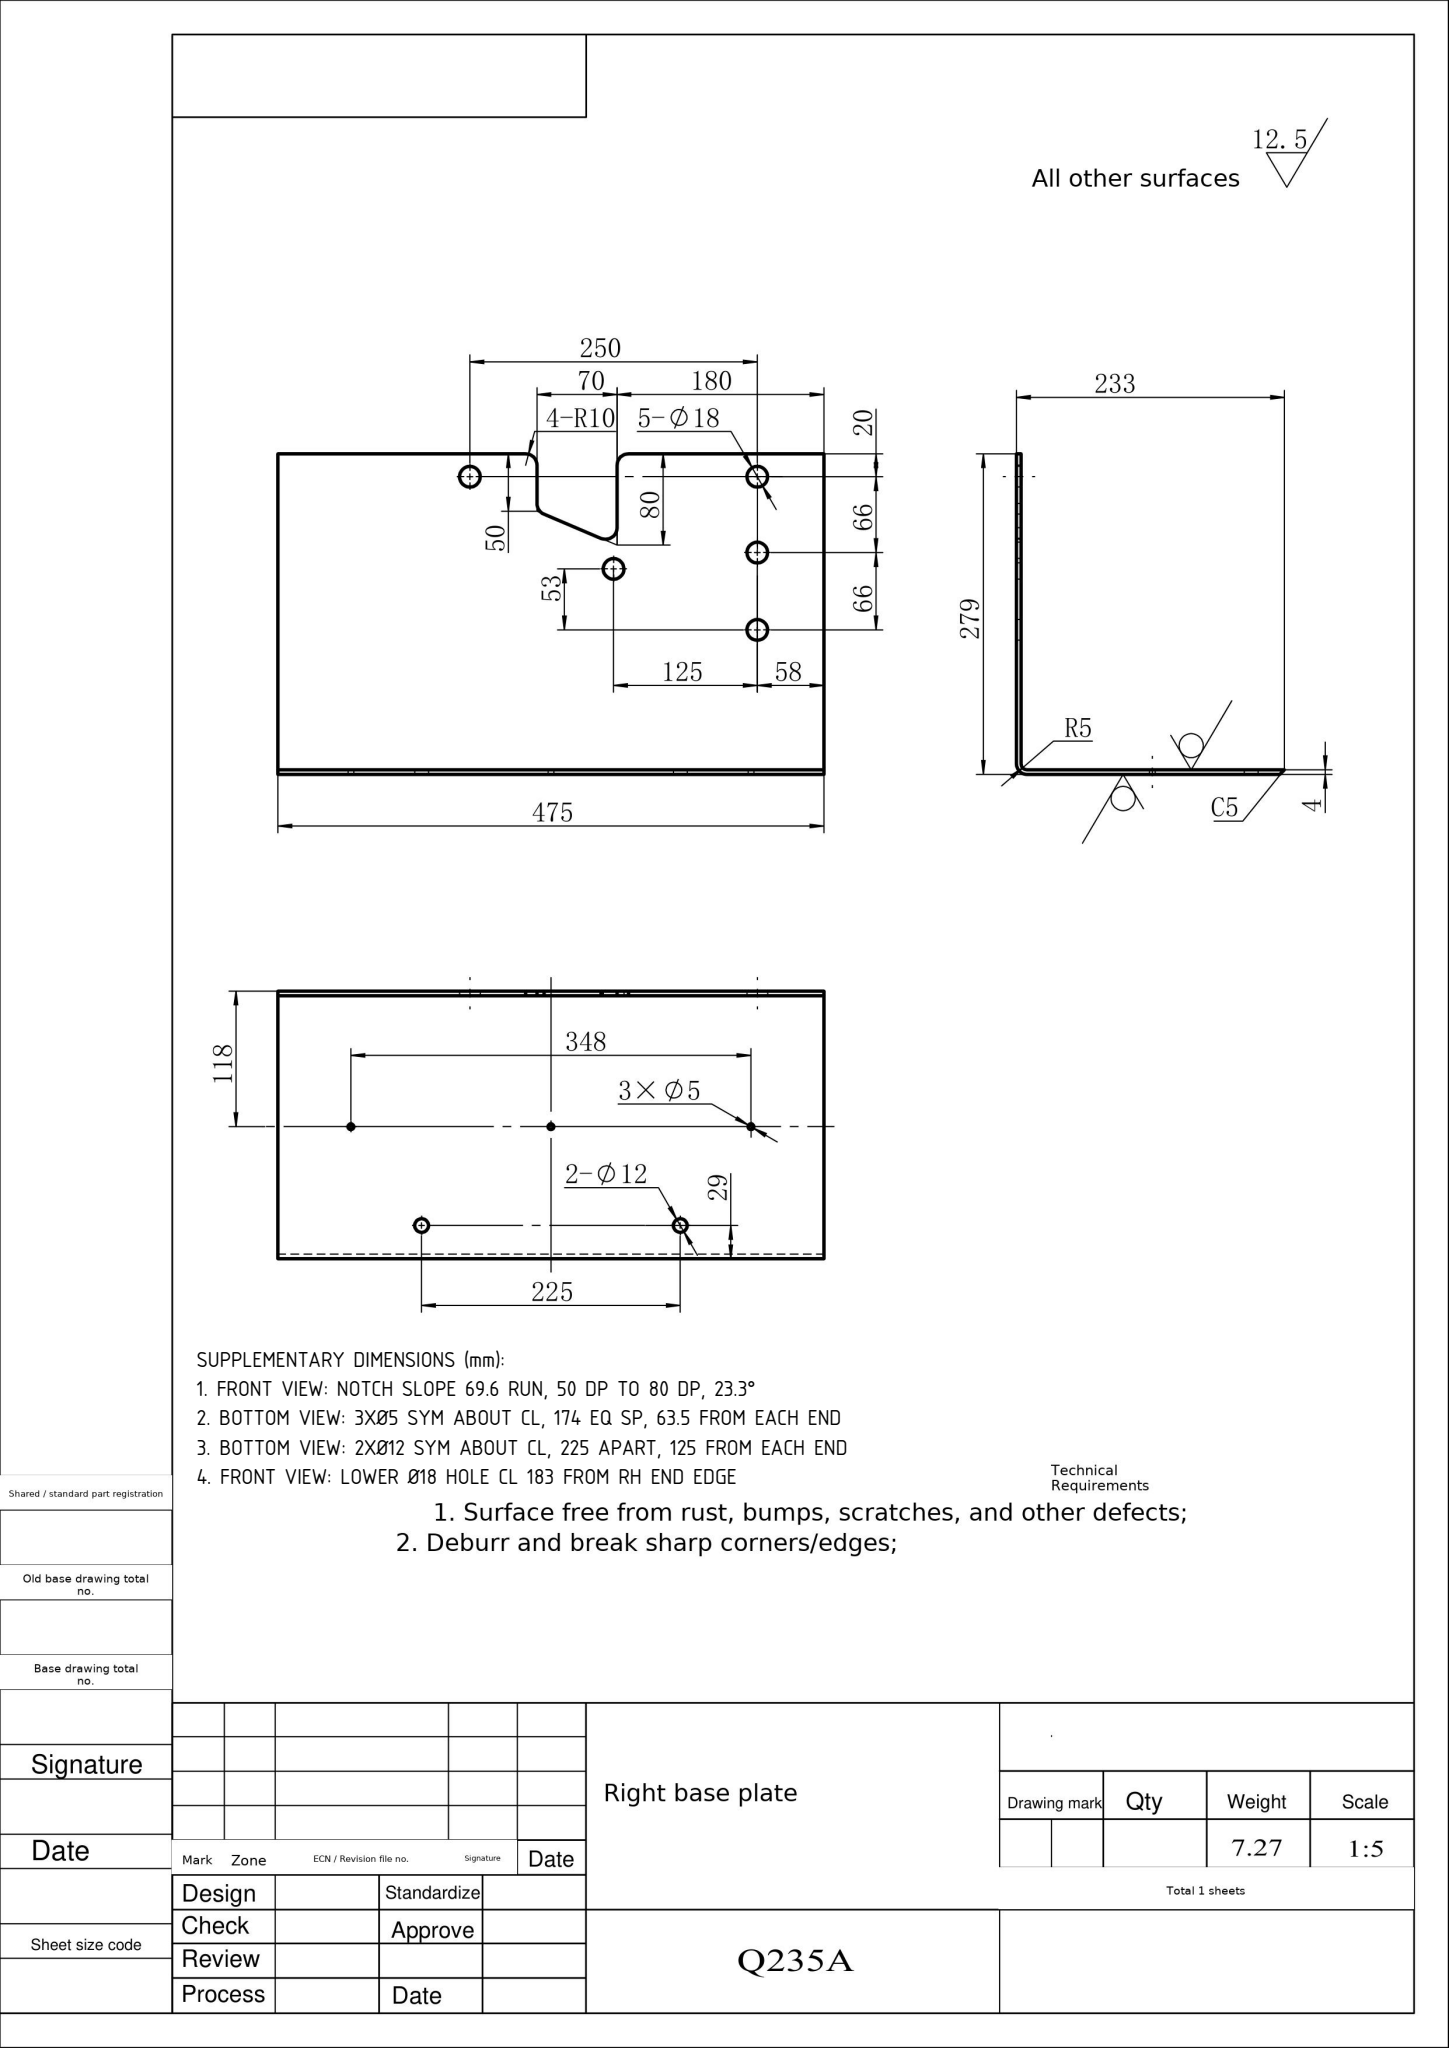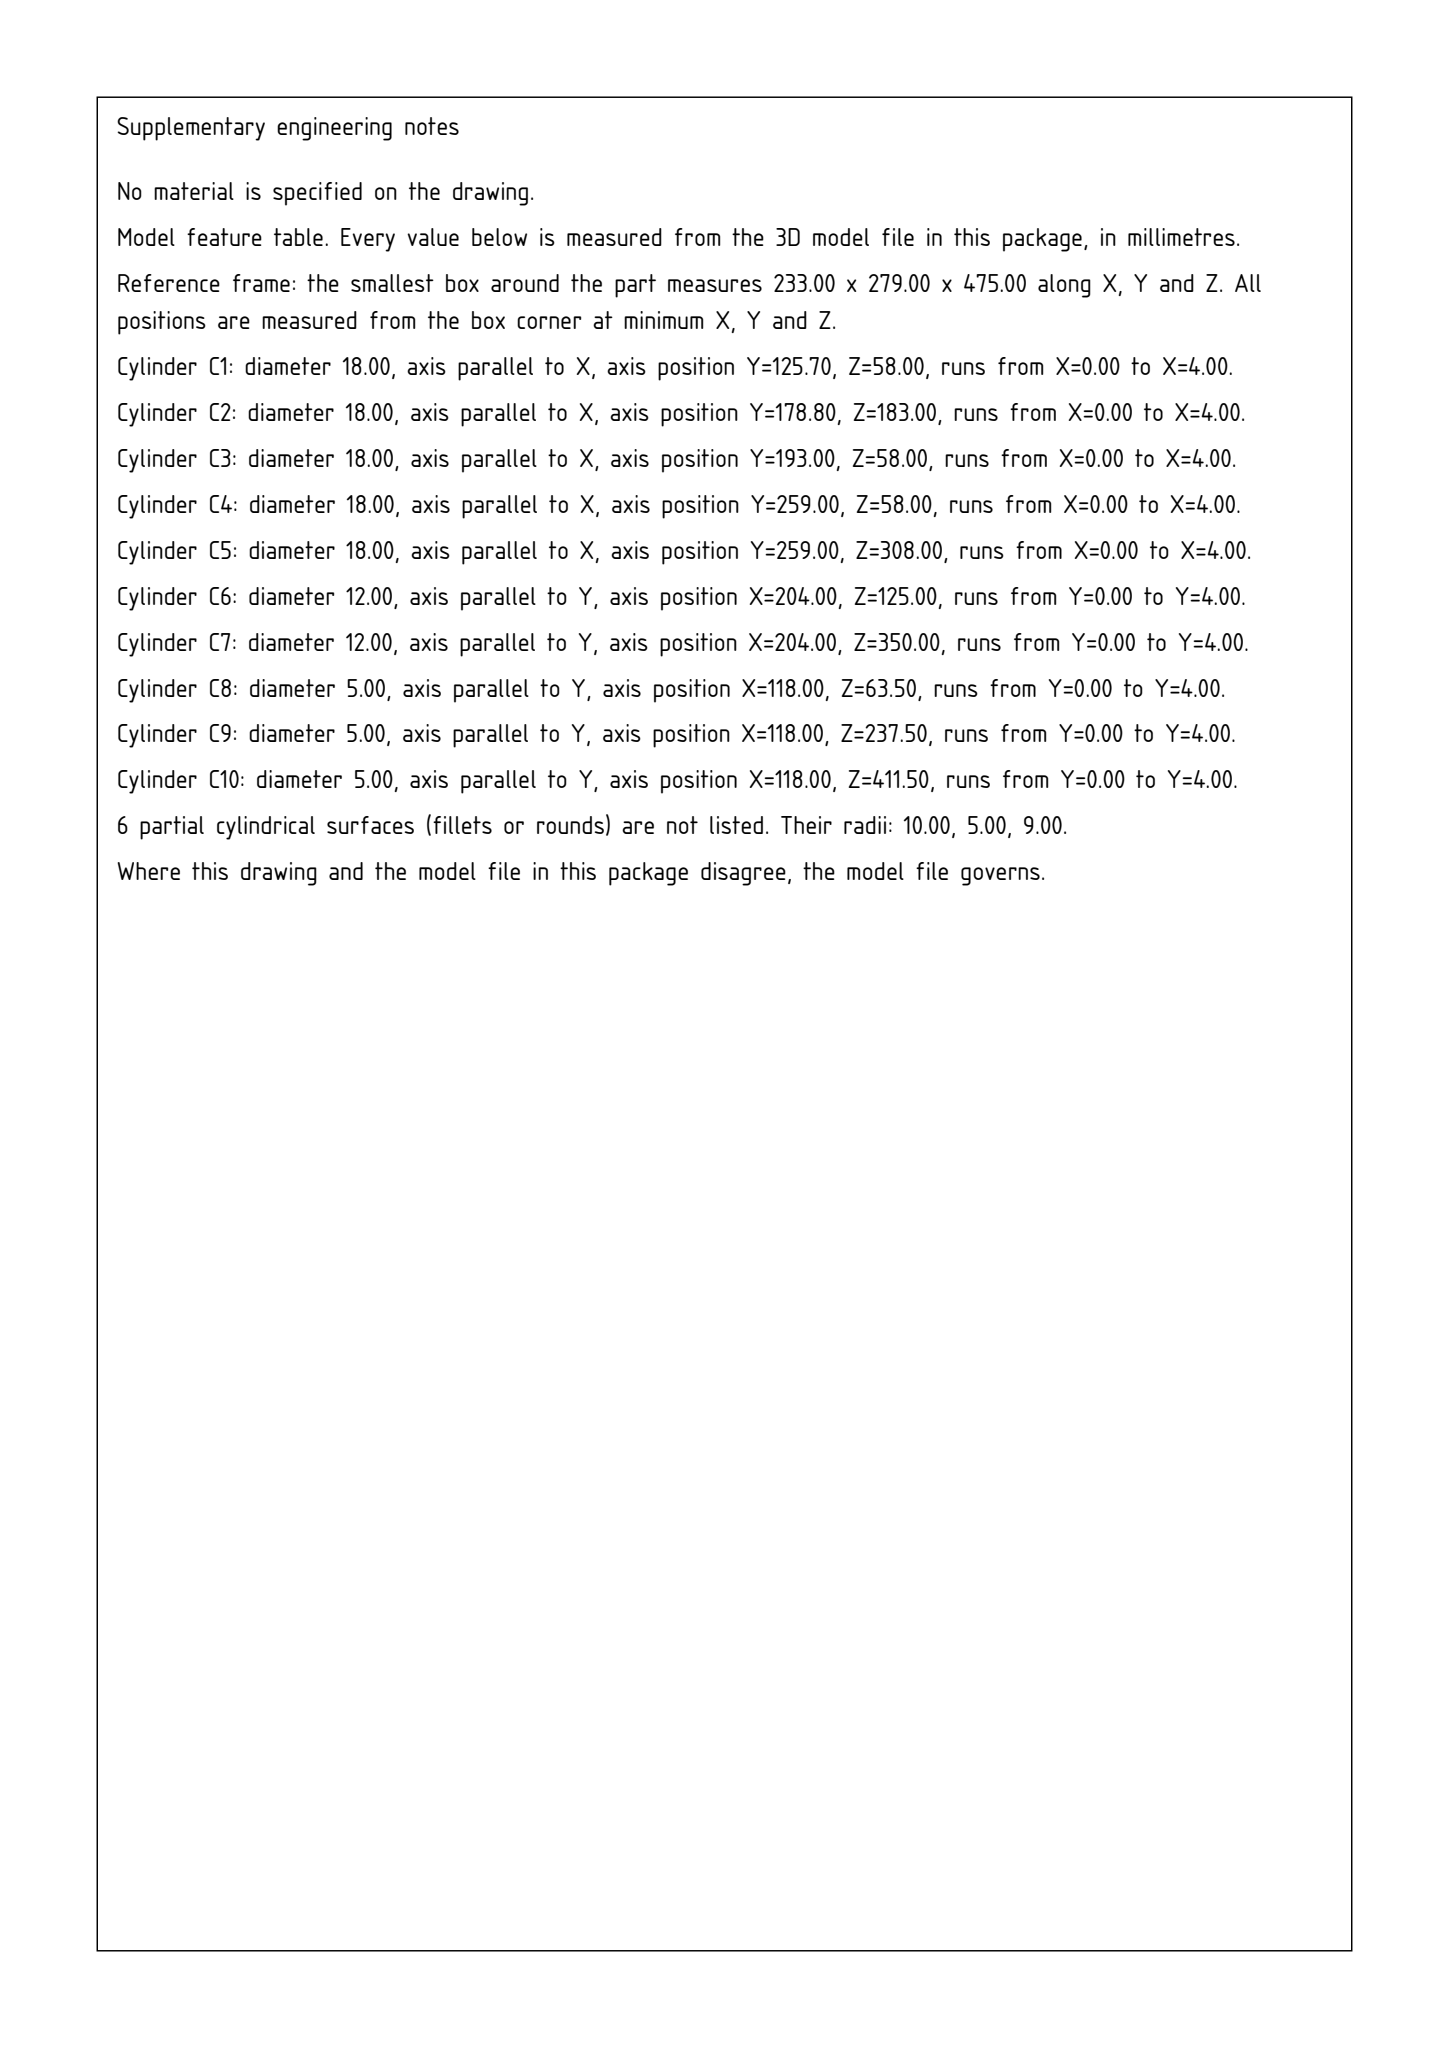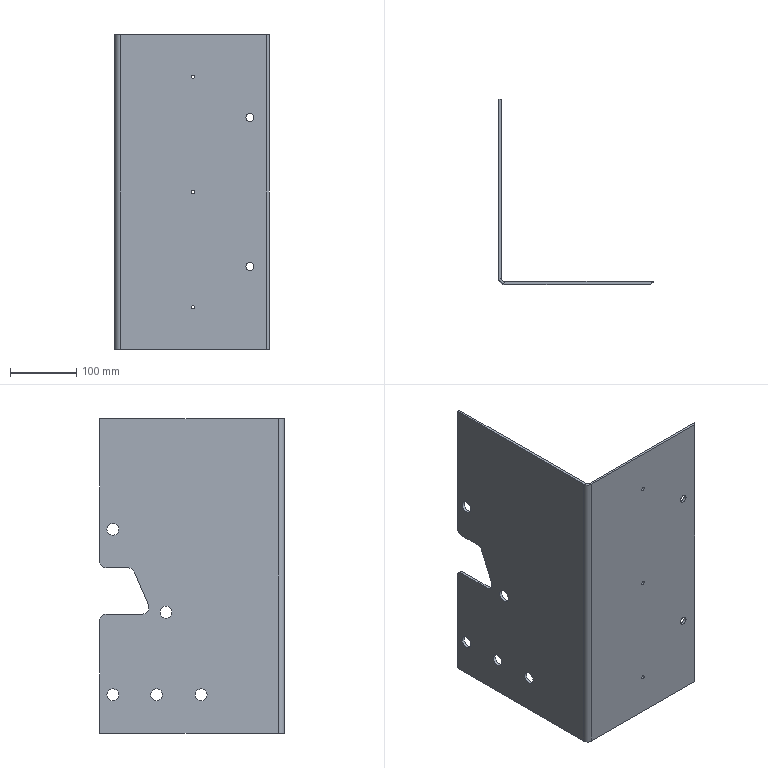Part | SolidWorks | mm | 1 solid | 43 faces | box 233 x 279 x 475 mm | volume 931498 mm3 | cylinder 27 | plane 16 | commonest cylinder face diameters 18 x11 5 x6 20 x5 12 x4 10 x1